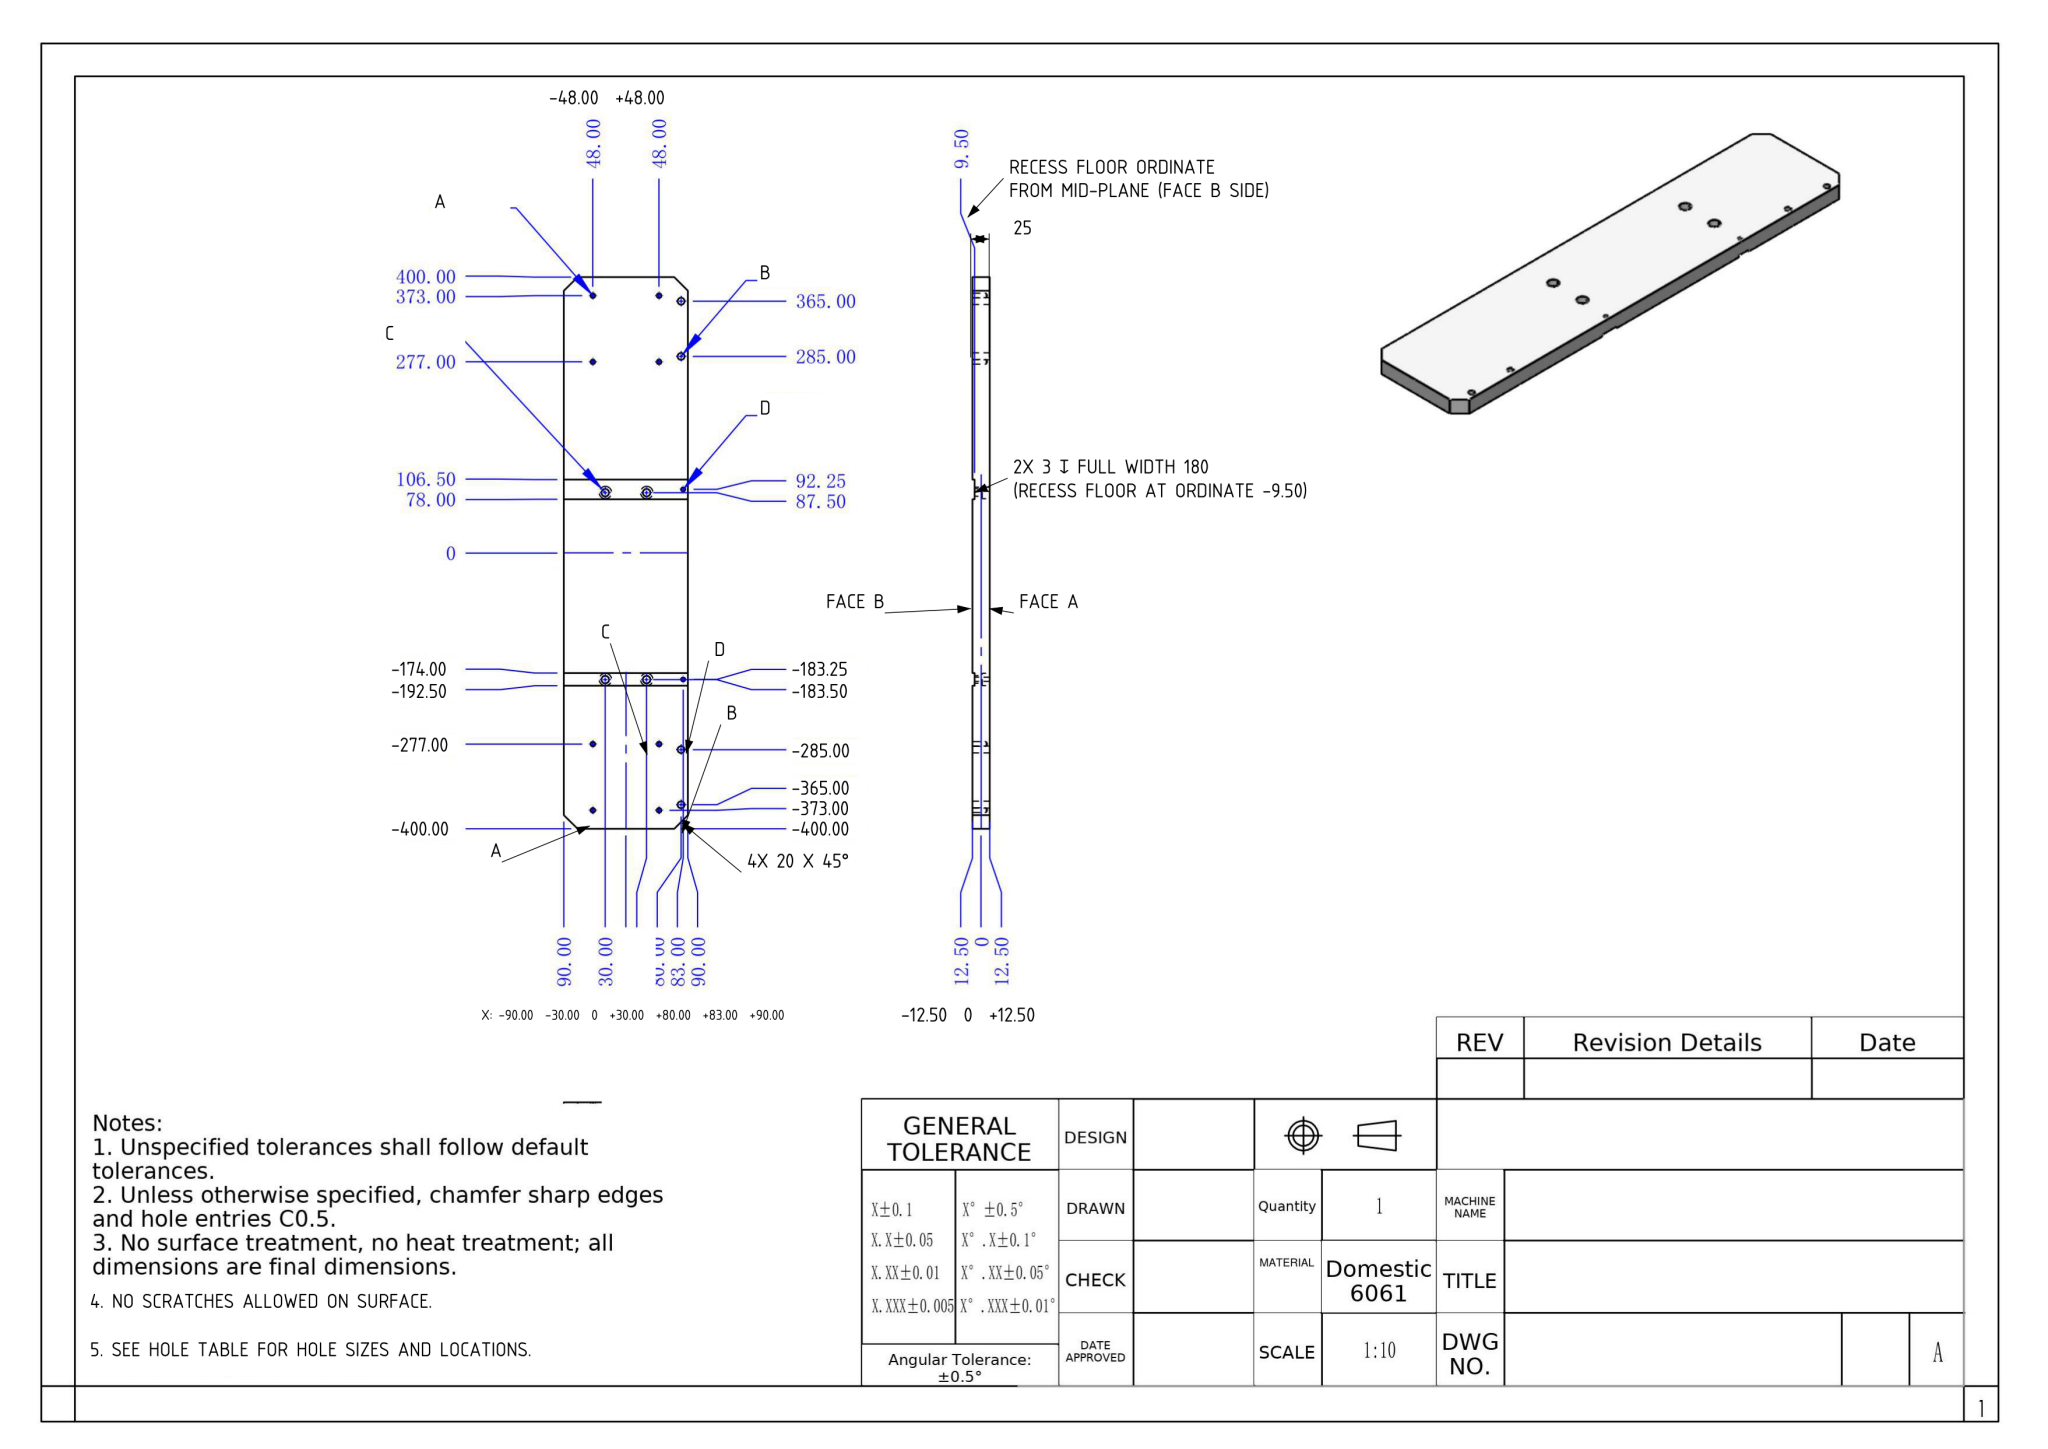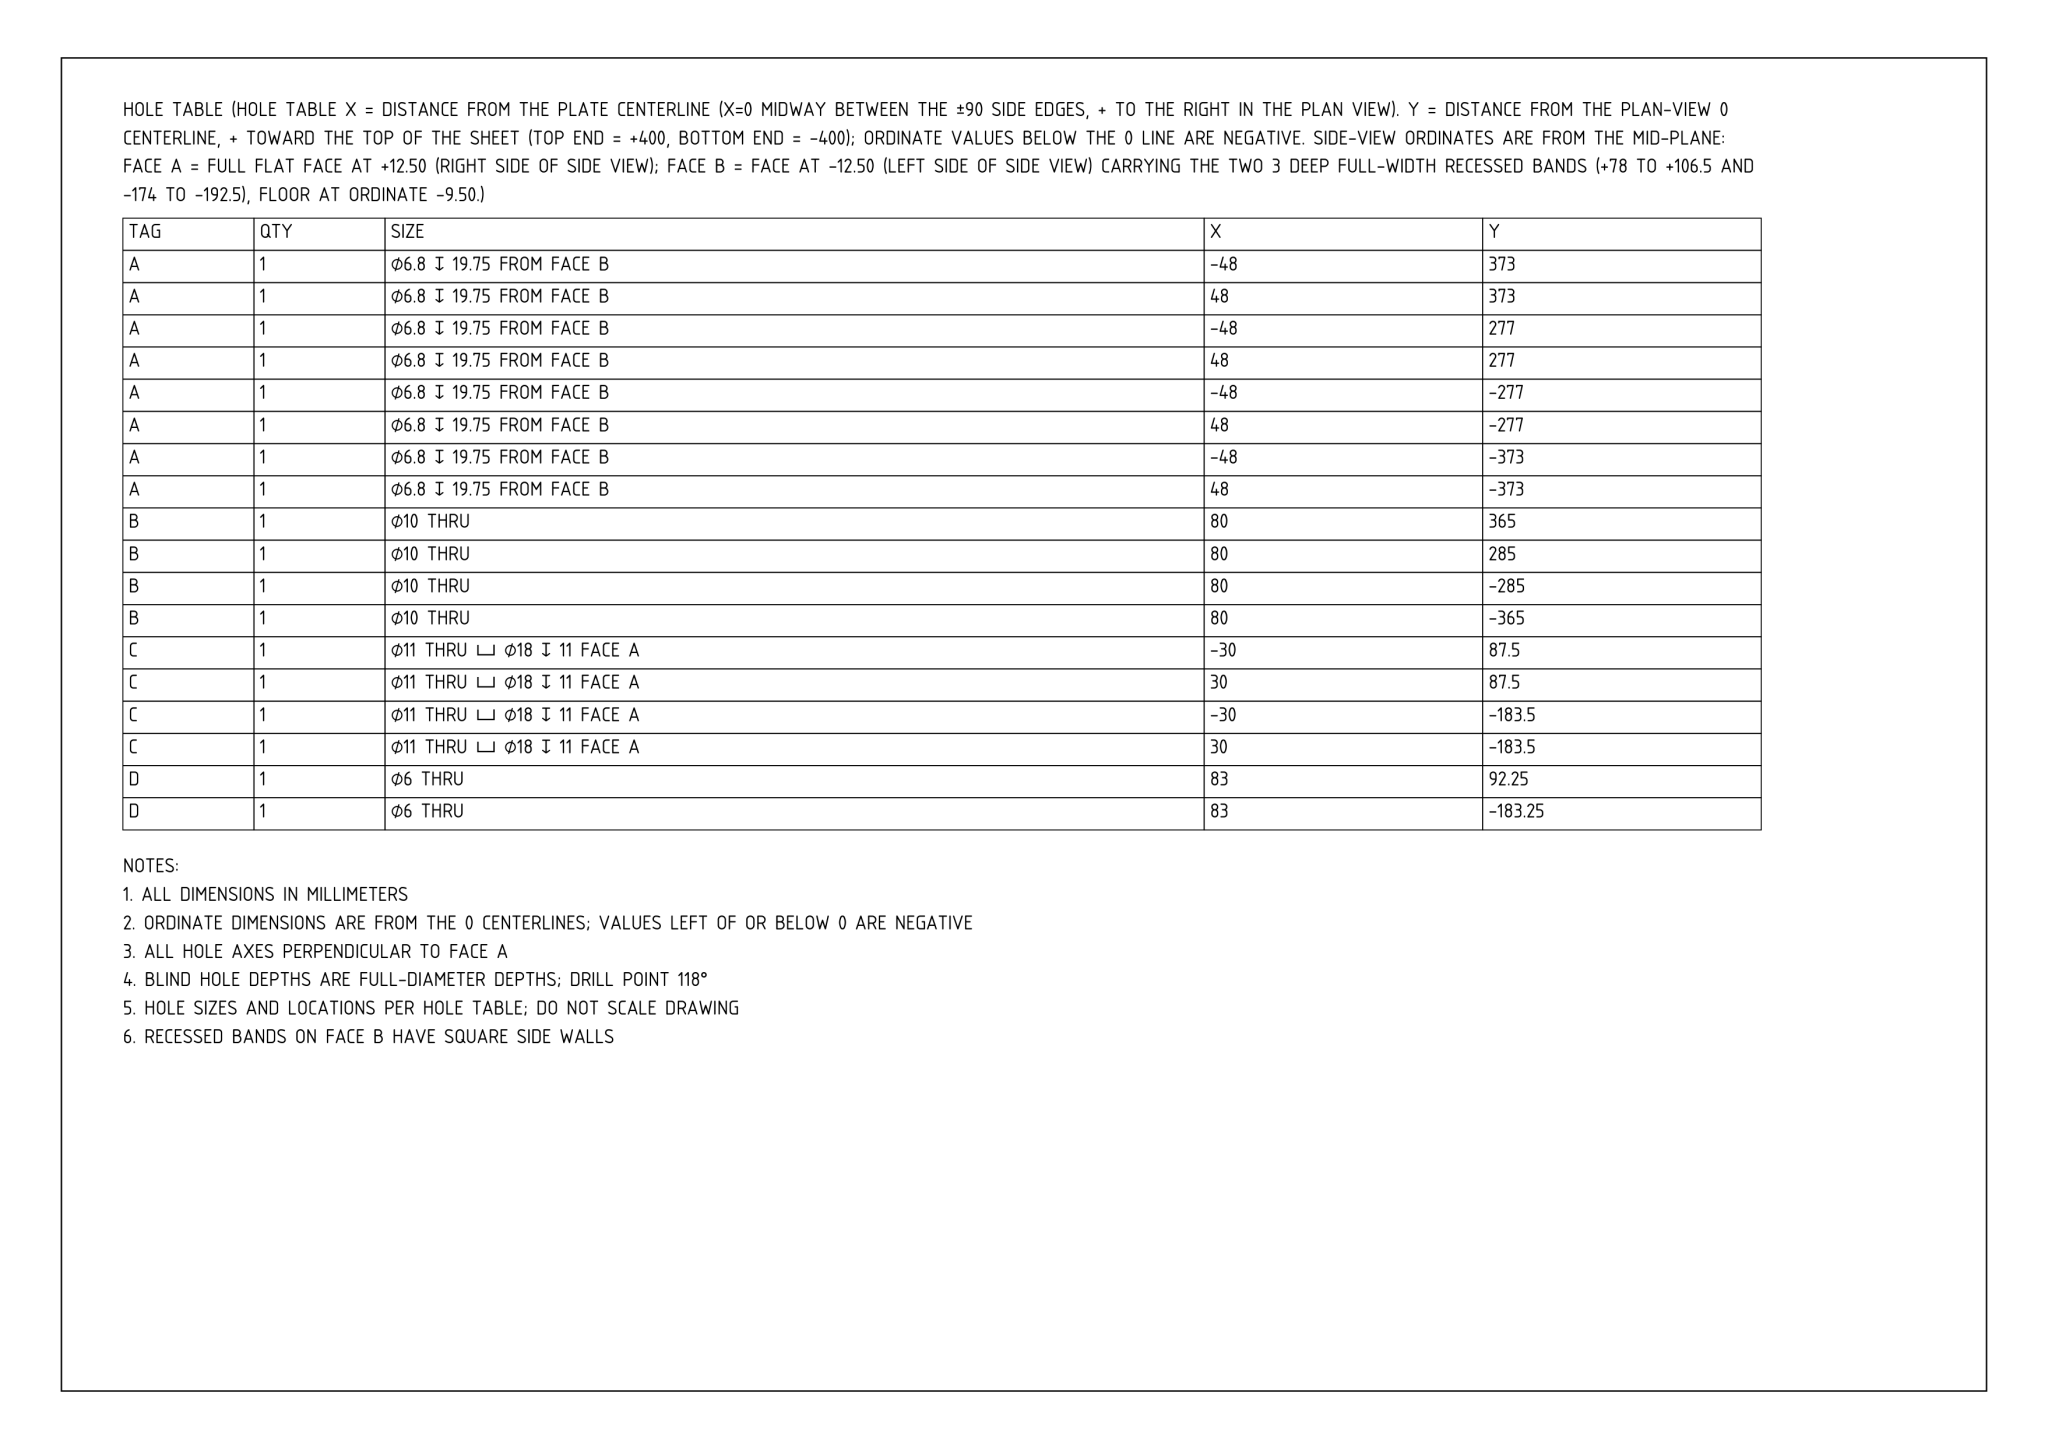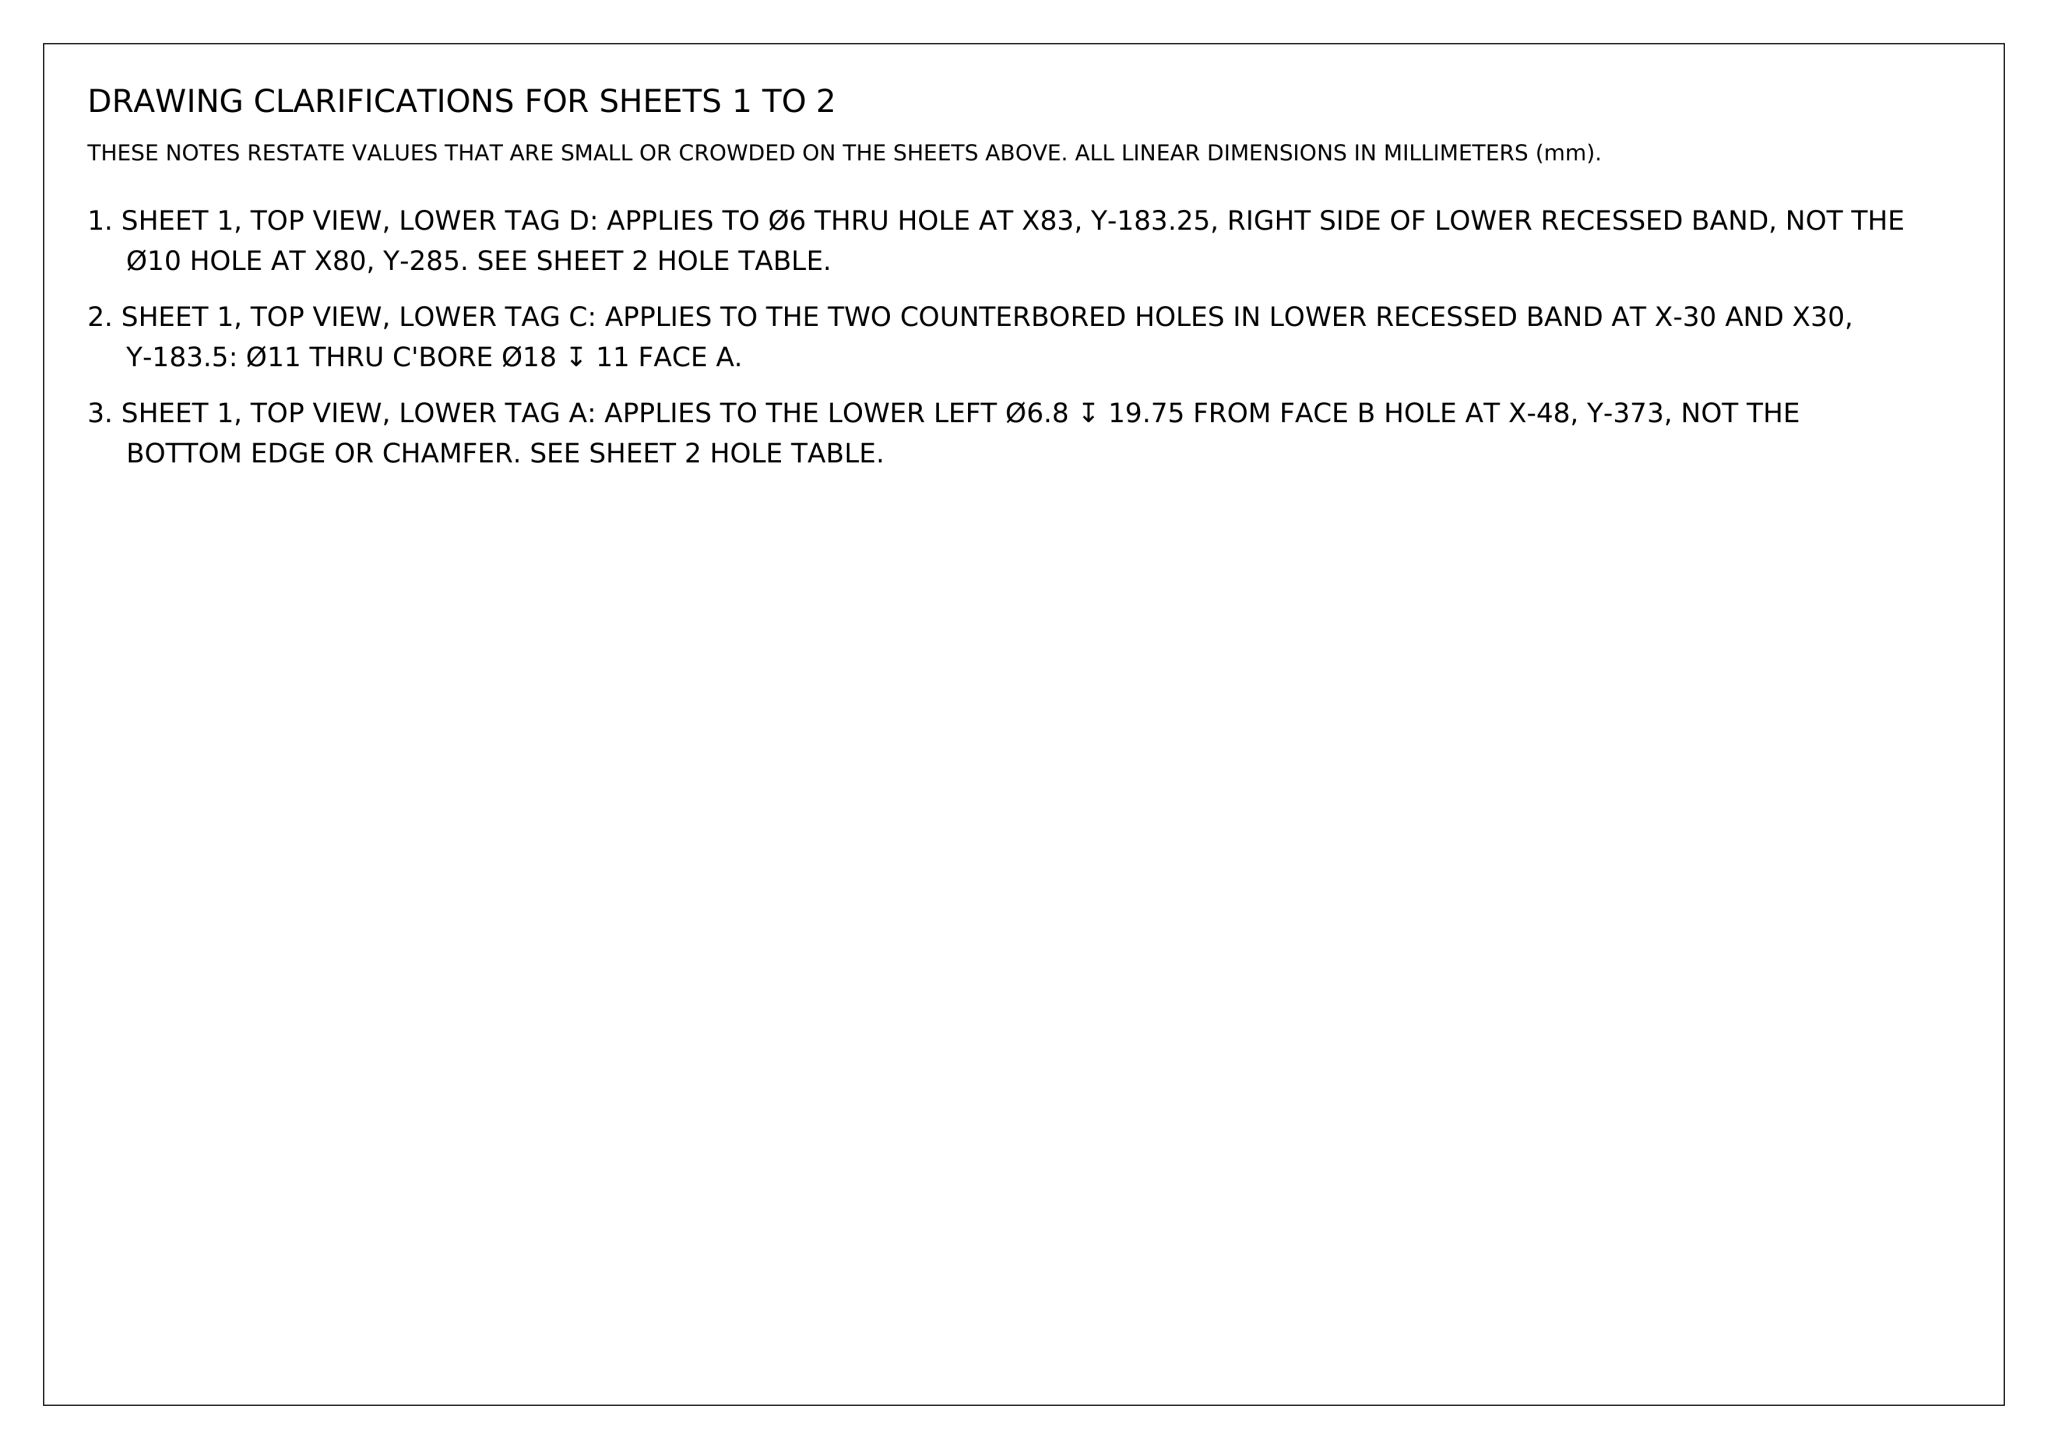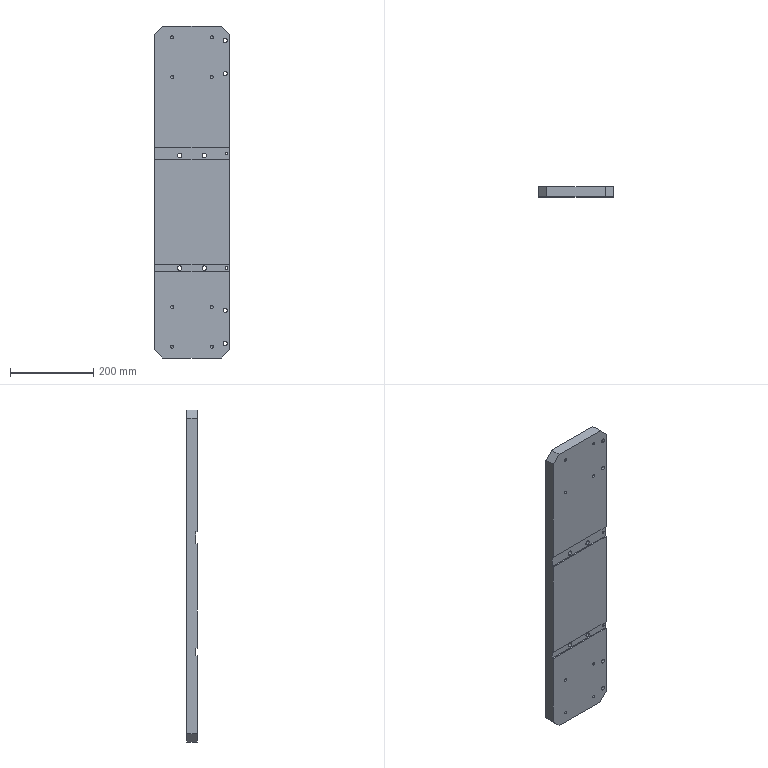Part | NX | mm | 1 solid | 82 faces | box 180 x 25 x 800 mm | volume 3524208 mm3 | cylinder 44 | plane 22 | cone 16 | commonest cylinder face diameters 6.8 x16 10 x8 18 x8 11 x8 6 x4